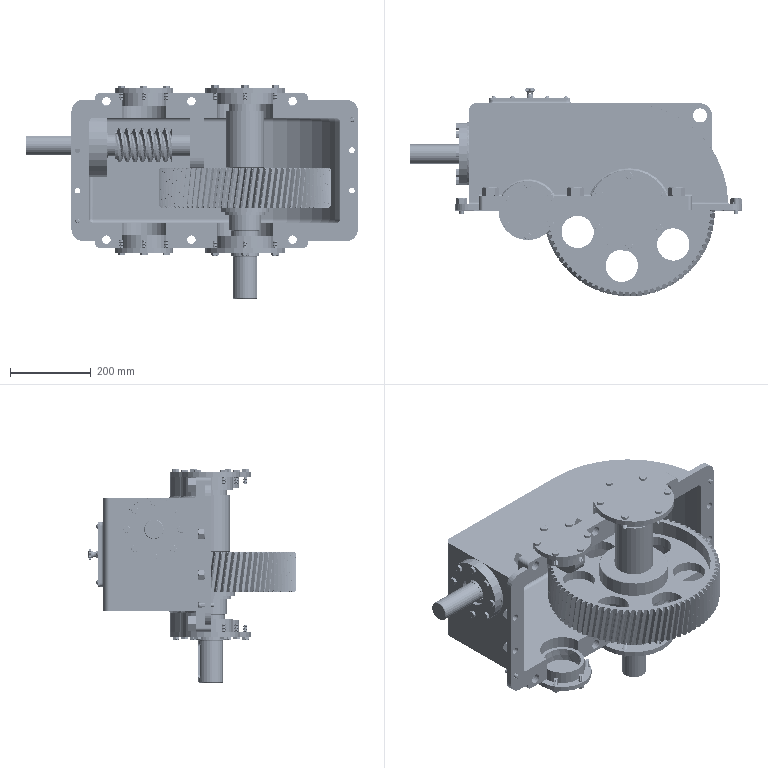Assembly | SolidWorks | mm | 84 component files | 84 solids | 4890 faces | box 820.25 x 516.08 x 527.4 mm | volume 19904523 mm3 | cylinder 2303 | plane 1060 | cone 558 | spline 498 | torus 360 | sphere 111 | commonest cylinder face diameters 10 x1442 0.5 x153 25 x112 20.75 x96 424.15 x83 6.708 x48 13 x27 11 x24
Bill of materials:
M10-30Bolt1 | 24 |  | Hex-head bolt-like part: hexagonal head with a short plain neck/undercut, then a long cylindrical shank with helical thread form to a flat end.
m16 | 4 |  | Tall hexagonal nut-like body with a central round through-bore and chamfered (arc-edged) hex corners at both ends.
M24 | 6 |  | Tall hexagonal nut-like body with a central threaded through-bore and chamfered hex corners at both ends.
FlangeOnLowSpeedAxis1 | 1 |  | Solid circular plate/blind flange with six through-holes on a bolt circle and a smaller-diameter raised cylindrical spigot on one face; no center bore.
FlangeOnLowSpeedAxis2 | 1 |  | Annular flange with six bolt holes and a raised cylindrical collar; the collar has a counterbore and a smaller central through-bore, forming an internal step.
FlangeOnWormWheelAxis | 2 |  | Cup-shaped flanged part: circular flange with six bolt holes supporting a tall cylindrical wall that encloses a recess with a closed bottom.
InvoluteLargeGear | 1 | Brass | Helical spur-type gear with many fine teeth, a recessed web containing six round lightening holes, a raised central hub, and a keyed central bore.
KeyOnLargeGear | 1 | Plain Carbon Steel | Small rectangular bar with fully rounded ends (obround/stadium plan shape) and small edge chamfers, resembling a round-ended parallel key.
LowSpeedAxis | 1 |  | Stepped cylindrical shaft with several coaxial diameter steps, largest step near one end with a short smaller pilot at that end, decreasing in diameter toward the other end.
SleeveOnLowSpeedAxis | 1 |  | Flat ring/washer with a stepped outer profile: a wider thin ring plus a slightly smaller-diameter thin step on one face, with a large central bore and small edge chamfers.
tapered roller bearings gb | 4 |  | Rolling-element bearing-like assembly: outer ring, inner ring and a single row of cylindrical rollers between them; inner ring protrudes axially on one side.
TaperPin | 2 |  | Solid tapered cylindrical pin, slightly larger diameter at one end, with chamfered edges at both ends.
circlips for holes--type a gb | 1 |  | Flat, thin open ring (C-shape) with uniform thickness. The two free ends widen into lugs, and each lug has a small round through-hole. Its form matches an internal-style retaining ring with lug holes.
FlangeOnWormAxis | 1 |  | Circular flat flange disc with a large central bore. It has eight equally spaced through-holes on a bolt circle and a short raised annular boss or face around the bore on one side.
hexagon socket button head screws gb | 6 |  | Solid pin with a domed (round) head and a plain cylindrical shank with a flat end. It has the shape of a solid round-head rivet blank.
M10-45 | 8 |  | Hex-head bolt. The shank is partly threaded, with a plain unthreaded section near the head and a short reduced-diameter neck directly under the head.
PeepHoleCover | 1 |  | Thin flat rectangular plate with rounded corners and nine through-holes: three across the top, three across the bottom, two at the mid-height side edges and one at the centre.
UpperHousing | 1 |  | Hollow, open-topped box-like housing with a perimeter mounting flange. Two side walls each have two semicircular bore cutouts with small holes around them, one end wall is curved, there is a rectangular opening with four holes in the floor, and an external lug has a single hole.
VentCap | 1 |  | Turned knob. It has a knurled, domed-top head, a concave waisted neck with a transverse cross-hole, a short collar and a smaller cylindrical spigot with a small axial bore at the end.
BearingSleeveOnWormAxis | 1 |  | Flanged tubular sleeve: a thin flat circular flange with eight equally spaced holes, joined to a short thin-walled cylindrical tube with a slight chamfer at its free end.
BearingInnerRing | 1 |  | Thick cylindrical ring or bush with a single external circumferential groove of rounded (concave) profile at about mid-width, and a plain cylindrical bore.
BearingOuterRing | 1 |  | Plain thin-walled cylindrical ring or band with slightly rounded or chamfered edges and a large bore.
Cage | 1 |  | Circular array of about 14 short ring-shaped loops, each joined to the next by small straight bar segments, forming a closed band.
RollingElement | 12 |  | Plain solid sphere.
WormAxis | 1 |  | Stepped cylindrical shaft with a short section of coarse helical thread (worm-like) between a long plain shank on one end and a short stepped journal on the other end.
Mates:
1. coincident | assembly face at (745.83, 1268.591, 1772.217) dir (0, 1, 0) | UpperHousingAssembly-1/UpperHousing-1 face at (890.83, 1268.591, 1632.217) dir (0, -1, 0)
2. concentric | assembly face at (798.33, 1008.59, 1803.217) dir (0, 1, 0) r 12.5 | UpperHousingAssembly-1/UpperHousing-1 face at (798.33, 1268.591, 1803.217) dir (0, 1, 0) r 12.5
3. concentric | UpperHousingAssembly-1/UpperHousing-1 face at (726.83, 1533.591, 1507.217) dir (0, -1, 0) r 6 | TaperPin-1 face at (726.83, 1299.341, 1507.217) dir (0, -1, 0) r 34.907
4. distance | TaperPin-1 face at (726.83, 1299.341, 1507.217) dir (0, 1, 0) | UpperHousingAssembly-1/UpperHousing-1 face at (890.83, 1283.591, 1632.217) dir (0, 1, 0)
5. concentric | UpperHousingAssembly-1/UpperHousing-1 face at (1404.83, 1533.591, 1757.217) dir (0, -1, 0) r 6 | TaperPin-2 face at (1404.83, 1299.341, 1757.217) dir (0, -1, 0) r 34.907
6. distance | TaperPin-2 face at (1404.83, 1299.341, 1757.217) dir (0, 1, 0) | UpperHousingAssembly-1/UpperHousing-1 face at (890.83, 1283.591, 1632.217) dir (0, 1, 0)
7. coincident | UpperHousingAssembly-1/UpperHousing-1 face at (890.83, 1303.591, 1632.217) dir (0, 1, 0) | M24-2 face at (1008.33, 1303.591, 1803.217) dir (0, -1, 0)
8. concentric | assembly face at (1258.33, 1008.59, 1461.217) dir (0, 1, 0) r 12.5 | assembly face at (798.33, 1453.938, 1461.217) dir (0, -1, 0) r 12
9. parallel | assembly face at (798.33, 1008.59, 1461.217) dir (0, 1, 0) r 12.5 | assembly face at (798.33, 1453.938, 1461.217) dir (0, -1, 0) r 12
10. concentric | assembly face at (798.33, 1008.59, 1461.217) dir (0, 1, 0) r 12.5 | assembly face at (798.33, 1453.938, 1461.217) dir (0, -1, 0) r 12
11. coincident | UpperHousingAssembly-1/UpperHousing-1 face at (890.83, 1303.591, 1632.217) dir (0, 1, 0) | M24-4 face at (1258.33, 1303.591, 1803.217) dir (0, -1, 0)
12. coincident | UpperHousingAssembly-1/UpperHousing-1 face at (890.83, 1303.591, 1632.217) dir (0, 1, 0) | M24-5 face at (798.33, 1303.591, 1461.217) dir (0, -1, 0)
13. coincident | UpperHousingAssembly-1/UpperHousing-1 face at (890.83, 1303.591, 1632.217) dir (0, 1, 0) | M24-7 face at (1258.33, 1303.591, 1461.217) dir (0, -1, 0)
14. coincident | UpperHousingAssembly-1/UpperHousing-1 face at (890.83, 1303.591, 1632.217) dir (0, 1, 0) | M24-6 face at (1008.33, 1303.591, 1461.217) dir (0, -1, 0)
15. concentric | PartAssemblyInLowerHousing-1/FlangeOnLowSpeedAxis2-1 face at (1140.83, 1354.591, 1428.217) dir (0, 0, 1) r 6.5 | M10-30Bolt1-1 face at (1140.83, 1354.591, 1458.217) dir (0, 0, 1) r 3.354
16. coincident | PartAssemblyInLowerHousing-1/FlangeOnLowSpeedAxis2-1 face at (1140.83, 1268.591, 1428.217) dir (0, 0, -1) | M10-30Bolt1-1 face at (1140.83, 1354.591, 1428.217) dir (0, 0, 1)
17. concentric | PartAssemblyInLowerHousing-1/FlangeOnWormWheelAxis-1 face at (890.83, 1332.591, 1429.217) dir (0, 0, 1) r 5.5 | M10-30Bolt1-7 face at (890.83, 1332.591, 1459.217) dir (0, 0, 1) r 3.354
18. coincident | PartAssemblyInLowerHousing-1/FlangeOnWormWheelAxis-1 face at (890.83, 1268.591, 1429.217) dir (0, 0, -1) | M10-30Bolt1-7 face at (890.83, 1332.591, 1429.217) dir (0, 0, 1)
19. concentric | PartAssemblyInLowerHousing-1/FlangeOnLowSpeedAxis1-1 face at (1140.83, 1354.591, 1797.467) dir (0, 0, 1) r 6.5 | M10-30Bolt1-13 face at (1140.83, 1354.591, 1806.217) dir (0, 0, -1) r 3.354
20. coincident | PartAssemblyInLowerHousing-1/FlangeOnLowSpeedAxis1-1 face at (1054.227, 1318.591, 1836.217) dir (0, 0, 1) | M10-30Bolt1-13 face at (1140.83, 1354.591, 1836.217) dir (0, 0, -1)
21. concentric | PartAssemblyInLowerHousing-1/FlangeOnWormWheelAxis-2 face at (890.83, 1332.591, 1835.217) dir (0, 0, -1) r 5.5 | M10-30Bolt1-25 face at (890.83, 1332.591, 1805.217) dir (0, 0, -1) r 3.354
22. coincident | PartAssemblyInLowerHousing-1/FlangeOnWormWheelAxis-2 face at (890.83, 1268.591, 1835.217) dir (0, 0, 1) | M10-30Bolt1-25 face at (890.83, 1332.591, 1835.217) dir (0, 0, -1)
23. coincident | UpperHousingAssembly-1/UpperHousing-1 face at (890.83, 1283.591, 1632.217) dir (0, 1, 0) | m16-2 face at (726.83, 1283.591, 1582.217) dir (0, -1, 0)
24. coincident | UpperHousingAssembly-1/UpperHousing-1 face at (890.83, 1283.591, 1632.217) dir (0, 1, 0) | m16-3 face at (726.83, 1283.591, 1682.217) dir (0, -1, 0)
25. coincident | UpperHousingAssembly-1/UpperHousing-1 face at (890.83, 1283.591, 1632.217) dir (0, 1, 0) | m16-4 face at (1404.83, 1283.591, 1682.217) dir (0, -1, 0)
26. coincident | UpperHousingAssembly-1/UpperHousing-1 face at (890.83, 1283.591, 1632.217) dir (0, 1, 0) | m16-5 face at (1404.83, 1283.591, 1582.217) dir (0, -1, 0)
27. concentric | LowSpeedAxisAssembly-1/tapered roller bearings gb-4 face at (1221.289, 1355.939, 1464.523) dir (0, 0, -1) r 32.5 | FlangeOnLowSpeedAxis1-1 face at (1221.289, 1355.939, 1508.526) dir (0, 0, 1) r 34.907
28. coincident | LowSpeedAxisAssembly-1/tapered roller bearings gb-4 face at (1192.973, 1369.74, 1482.776) dir (0, 0, 1) | FlangeOnLowSpeedAxis1-1 face at (1167.596, 1386.939, 1482.776) dir (0, 0, -1)
29. coincident | LowSpeedAxis-1 face at (1124.62, 1130.298, 1182.59) dir (0, 1, 0) | KeyOnLargeGear-1 face at (1059.62, 1130.298, 1182.59) dir (0, -1, 0)
30. concentric | LowSpeedAxis-1 face at (1124.62, 1130.298, 1182.59) dir (0, 1, 0) r 11 | KeyOnLargeGear-1 face at (1124.62, 1130.298, 1182.59) dir (0, 1, 0) r 11
31. coincident | KeyOnLargeGear-1 face at (1059.62, 1130.298, 1193.59) dir (0, 0, 1) | InvoluteLargeGear-1 face at (1139.626, 1137.849, 1193.59) dir (0, 0, -1)
32. coincident | LowSpeedAxis-1 face at (1139.62, 1139.298, 1182.59) dir (-1, 0, 0) | InvoluteLargeGear-1 face at (1139.62, 1096.798, 1182.59) dir (1, 0, 0)
33. concentric | LowSpeedAxis-1 face at (805.297, 1096.798, 1182.59) dir (-1, 0, 0) r 40 | SleeveOnLowSpeedAxis-1 face at (1039.62, 1096.798, 1182.59) dir (1, 0, 0) r 40
34. coincident | InvoluteLargeGear-1 face at (1039.62, 1096.798, 1182.59) dir (-1, 0, 0) | SleeveOnLowSpeedAxis-1 face at (1039.62, 1087.814, 1241.914) dir (1, 0, 0)
35. concentric | LowSpeedAxis-1 face at (805.297, 1096.798, 1182.59) dir (-1, 0, 0) r 40 | tapered roller bearings gb-3 face at (1021.87, 1096.798, 1182.59) dir (1, 0, 0) r 16
36. coincident | SleeveOnLowSpeedAxis-1 face at (1021.87, 1090.809, 1222.139) dir (-1, 0, 0) | tapered roller bearings gb-3 face at (1021.87, 1096.798, 1182.59) dir (1, 0, 0)
37. concentric | LowSpeedAxis-1 face at (805.297, 1096.798, 1182.59) dir (-1, 0, 0) r 40 | tapered roller bearings gb-4 face at (1279.62, 1096.798, 1182.59) dir (-1, 0, 0) r 16
38. coincident | LowSpeedAxis-1 face at (1279.62, 1144.298, 1182.59) dir (1, 0, 0) | tapered roller bearings gb-4 face at (1279.62, 1096.798, 1182.59) dir (-1, 0, 0)
39. concentric | LowSpeedAxis-1 face at (805.297, 1096.798, 1182.59) dir (-1, 0, 0) r 42.5 | InvoluteLargeGear-1 face at (1139.626, 1096.798, 1182.59) dir (-1, 0, 0) r 42.5
40. concentric | UpperHousing-1 face at (835.485, 1282.284, 1275.253) dir (1, 0, 0) r 50 | circlips for holes--type a gb-1 face at (1154.736, 1282.284, 1275.253) dir (1, 0, 0) r 6.5
41. coincident | UpperHousing-1 face at (1154.736, 1282.284, 1328.003) dir (1, 0, 0) | circlips for holes--type a gb-1 face at (1154.736, 1282.284, 1275.253) dir (-1, 0, 0)
42. concentric | UpperHousing-1 face at (864.486, 1282.284, 1275.253) dir (-1, 0, 0) r 55 | WormAxisAssembly-1/BearingSleeveOnWormAxis-1 face at (920.486, 1282.284, 1275.253) dir (-1, 0, 0) r 55
43. concentric | UpperHousing-1 face at (864.486, 1349.284, 1275.253) dir (-1, 0, 0) r 5 | WormAxisAssembly-1/BearingSleeveOnWormAxis-1 edge at (855.486, 1349.284, 1275.253) dir (-1, 0, 0) r 5.275
44. coincident | UpperHousing-1 face at (864.486, 1282.284, 1275.253) dir (-1, 0, 0) | WormAxisAssembly-1/BearingSleeveOnWormAxis-1 face at (864.486, 1282.284, 1275.253) dir (1, 0, 0)
45. coincident | WormAxisAssembly-1/BearingSleeveOnWormAxis-1 face at (855.486, 1282.284, 1275.253) dir (-1, 0, 0) | FlangeOnWormAxis-1 face at (855.486, 1360.284, 1275.253) dir (1, 0, 0)
46. concentric | WormAxisAssembly-1/WormAxis-1 face at (723.233, 1282.284, 1275.253) dir (-1, 0, 0) r 24 | FlangeOnWormAxis-1 face at (843.486, 1282.284, 1275.253) dir (-1, 0, 0) r 78
47. concentric | UpperHousing-1 face at (864.486, 1329.66, 1322.629) dir (-1, 0, 0) r 5 | FlangeOnWormAxis-1 face at (861.986, 1329.66, 1322.629) dir (-1, 0, 0) r 5.25
48. coincident | UpperHousing-1 face at (1014.486, 1415.284, 1213.253) dir (0, 1, 0) | PeepHoleCover-1 face at (1019.486, 1415.284, 1213.253) dir (0, -1, 0)
49. concentric | UpperHousing-1 edge at (1061.986, 1415.284, 1282.253) dir (0, 1, 0) r 5 | PeepHoleCover-1 edge at (1061.986, 1421.284, 1282.253) dir (0, 1, 0) r 5
50. concentric | UpperHousing-1 edge at (930.486, 1415.284, 1213.253) dir (0, 1, 0) r 5 | PeepHoleCover-1 edge at (930.486, 1421.284, 1213.253) dir (0, 1, 0) r 5
51. concentric | PeepHoleCover-1 face at (1019.486, 1421.284, 1213.253) dir (0, 1, 0) r 5 | VentCap-1 face at (1019.486, 1411.284, 1213.253) dir (0, -1, 0) r 5
52. coincident | PeepHoleCover-1 face at (1019.486, 1421.284, 1213.253) dir (0, 1, 0) | VentCap-1 edge at (1019.486, 1421.284, 1213.253) dir (0, -1, 0) r 8
53. concentric | FlangeOnWormAxis-1 face at (861.986, 1349.284, 1275.253) dir (-1, 0, 0) r 5.25 | M10-45-1 face at (888.486, 1349.284, 1275.253) dir (1, 0, 0) r 3.092
54. coincident | FlangeOnWormAxis-1 face at (843.486, 1318.284, 1275.253) dir (-1, 0, 0) | M10-45-1 face at (843.486, 1349.284, 1275.253) dir (1, 0, 0)
55. concentric | FlangeOnWormAxis-1 face at (861.986, 1329.66, 1227.877) dir (-1, 0, 0) r 5.25 | M10-45-3 face at (888.486, 1329.66, 1227.877) dir (1, 0, 0) r 3.092
56. concentric | FlangeOnWormAxis-1 face at (861.986, 1282.284, 1208.253) dir (-1, 0, 0) r 5.25 | M10-45-6 face at (888.486, 1282.284, 1208.253) dir (1, 0, 0) r 3.092
57. concentric | FlangeOnWormAxis-1 edge at (843.486, 1329.66, 1322.629) dir (-1, 0, 0) r 5.25 | M10-45-7 face at (888.486, 1329.66, 1322.629) dir (1, 0, 0) r 3.092
58. concentric | FlangeOnWormAxis-1 face at (861.986, 1282.284, 1342.253) dir (-1, 0, 0) r 5.25 | M10-45-2 face at (888.486, 1282.284, 1342.253) dir (1, 0, 0) r 3.092
59. concentric | FlangeOnWormAxis-1 face at (861.986, 1234.908, 1227.877) dir (-1, 0, 0) r 5.25 | M10-45-4 face at (888.486, 1234.908, 1227.877) dir (1, 0, 0) r 3.092
60. concentric | FlangeOnWormAxis-1 face at (861.986, 1215.284, 1275.253) dir (-1, 0, 0) r 5.25 | M10-45-5 face at (888.486, 1215.284, 1275.253) dir (1, 0, 0) r 3.092
61. concentric | FlangeOnWormAxis-1 face at (861.986, 1234.908, 1322.629) dir (-1, 0, 0) r 5.25 | M10-45-8 face at (888.486, 1234.908, 1322.629) dir (1, 0, 0) r 3.092
62. coincident | FlangeOnWormAxis-1 face at (843.486, 1318.284, 1275.253) dir (-1, 0, 0) | M10-45-8 face at (843.486, 1234.908, 1322.629) dir (1, 0, 0)
63. coincident | FlangeOnWormAxis-1 face at (843.486, 1318.284, 1275.253) dir (-1, 0, 0) | M10-45-4 face at (843.486, 1234.908, 1227.877) dir (1, 0, 0)
64. coincident | FlangeOnWormAxis-1 face at (843.486, 1318.284, 1275.253) dir (-1, 0, 0) | M10-45-5 face at (843.486, 1215.284, 1275.253) dir (1, 0, 0)
65. coincident | FlangeOnWormAxis-1 face at (843.486, 1318.284, 1275.253) dir (-1, 0, 0) | M10-45-3 face at (843.486, 1329.66, 1227.877) dir (1, 0, 0)
66. coincident | FlangeOnWormAxis-1 face at (843.486, 1318.284, 1275.253) dir (-1, 0, 0) | M10-45-6 face at (843.486, 1282.284, 1208.253) dir (1, 0, 0)
67. coincident | FlangeOnWormAxis-1 face at (843.486, 1318.284, 1275.253) dir (-1, 0, 0) | M10-45-7 face at (843.486, 1329.66, 1322.629) dir (1, 0, 0)
68. coincident | FlangeOnWormAxis-1 face at (843.486, 1318.284, 1275.253) dir (-1, 0, 0) | M10-45-2 face at (843.486, 1282.284, 1342.253) dir (1, 0, 0)
69. concentric | PeepHoleCover-1 face at (1061.986, 1421.284, 1282.253) dir (0, 1, 0) r 5 | hexagon socket button head screws gb-8 face at (1061.986, 1401.284, 1282.253) dir (0, 1, 0) r 3
70. coincident | PeepHoleCover-1 face at (1019.486, 1421.284, 1213.253) dir (0, 1, 0) | hexagon socket button head screws gb-8 face at (1061.986, 1421.284, 1282.253) dir (0, -1, 0)
71. concentric | PeepHoleCover-1 face at (976.986, 1421.284, 1282.253) dir (0, 1, 0) r 5 | hexagon socket button head screws gb-9 face at (976.986, 1401.284, 1282.253) dir (0, 1, 0) r 3
72. coincident | PeepHoleCover-1 face at (1019.486, 1421.284, 1213.253) dir (0, 1, 0) | hexagon socket button head screws gb-9 face at (976.986, 1421.284, 1282.253) dir (0, -1, 0)
73. concentric | PeepHoleCover-1 face at (930.486, 1421.284, 1213.253) dir (0, 1, 0) r 5 | hexagon socket button head screws gb-10 face at (930.486, 1401.284, 1213.253) dir (0, 1, 0) r 3
74. coincident | PeepHoleCover-1 face at (1019.486, 1421.284, 1213.253) dir (0, 1, 0) | hexagon socket button head screws gb-10 face at (930.486, 1421.284, 1213.253) dir (0, -1, 0)
75. concentric | PeepHoleCover-1 face at (976.986, 1421.284, 1144.253) dir (0, 1, 0) r 5 | hexagon socket button head screws gb-11 face at (976.986, 1401.284, 1144.253) dir (0, 1, 0) r 3
76. coincident | PeepHoleCover-1 face at (1019.486, 1421.284, 1213.253) dir (0, 1, 0) | hexagon socket button head screws gb-11 face at (976.986, 1421.284, 1144.253) dir (0, -1, 0)
77. concentric | PeepHoleCover-1 face at (1061.986, 1421.284, 1144.253) dir (0, 1, 0) r 5 | hexagon socket button head screws gb-12 face at (1061.986, 1401.284, 1144.253) dir (0, 1, 0) r 3
78. coincident | PeepHoleCover-1 face at (1019.486, 1421.284, 1213.253) dir (0, 1, 0) | hexagon socket button head screws gb-12 face at (1061.986, 1421.284, 1144.253) dir (0, -1, 0)
79. concentric | PeepHoleCover-1 face at (1108.486, 1421.284, 1213.253) dir (0, 1, 0) r 5 | hexagon socket button head screws gb-13 face at (1108.486, 1401.284, 1213.253) dir (0, 1, 0) r 3
80. coincident | PeepHoleCover-1 face at (1019.486, 1421.284, 1213.253) dir (0, 1, 0) | hexagon socket button head screws gb-13 face at (1108.486, 1421.284, 1213.253) dir (0, -1, 0)
81. concentric | WormAxis-1 face at (855.062, 1105.253, 1134.051) dir (-1, 0, 0) r 22.5 | DeepGrooveBallBearing6309-1/BearingInnerRing-1 face at (1255.642, 1105.253, 1134.051) dir (-1, 0, 0) r 22.5
82. coincident | WormAxis-1 face at (1262.062, 1132.753, 1134.051) dir (1, 0, 0) | DeepGrooveBallBearing6309-1/BearingInnerRing-1 face at (1262.062, 1127.753, 1134.051) dir (-1, 0, 0)
83. concentric | tapered roller bearings gb-3 face at (1029.062, 1105.253, 1134.051) dir (-1, 0, 0) r 32.5 | tapered roller bearings gb-4 face at (1029.062, 1105.253, 1134.051) dir (1, 0, 0) r 32.5
84. coincident | tapered roller bearings gb-3 face at (1029.062, 1105.253, 1134.051) dir (-1, 0, 0) | tapered roller bearings gb-4 face at (1029.062, 1105.253, 1134.051) dir (1, 0, 0)
85. concentric | BearingSleeveOnWormAxis-1 face at (1047.315, 1105.253, 1134.051) dir (-1, 0, 0) r 50 | tapered roller bearings gb-4 face at (1029.062, 1105.253, 1134.051) dir (1, 0, 0) r 32.5
86. coincident | BearingSleeveOnWormAxis-1 face at (1047.315, 1105.253, 1134.051) dir (-1, 0, 0) | tapered roller bearings gb-3 face at (1047.315, 1135.278, 1143.576) dir (1, 0, 0)
87. concentric | WormAxis-1 face at (855.062, 1105.253, 1134.051) dir (-1, 0, 0) r 27.5 | BearingSleeveOnWormAxis-1 face at (1052.315, 1105.253, 1134.051) dir (-1, 0, 0) r 55
88. coincident | WormAxis-1 face at (1046.062, 1132.753, 1134.051) dir (-1, 0, 0) | tapered roller bearings gb-3 face at (1046.062, 1105.253, 1134.051) dir (1, 0, 0)
89. concentric | BearingInnerRing-1 face at (1013.335, 1022.594, 1021.051) dir (-1, 0, 0) r 22.5 | BearingOuterRing-1 face at (1026.403, 1022.594, 1021.051) dir (-1, 0, 0) r 50
90. coincident | BearingInnerRing-1 face at (1044.754, 1045.094, 1021.051) dir (1, 0, 0) | BearingOuterRing-1 face at (1044.754, 1072.594, 1021.051) dir (1, 0, 0)
91. coincident | BearingOuterRing-1 plane at (1032.254, 1022.594, 1021.051) dir (1, 0, 0) | Cage-1 plane at (1032.254, 1022.594, 1021.051) dir (1, 0, 0)
92. coincident | BearingInnerRing-1 axis at (1044.754, 1022.594, 1021.051) dir (-1, 0, 0) | Cage-1 axis at (1031.254, 1022.594, 1021.051) dir (1, 0, 0)
93. concentric | RollingElement-1 face at (1032.254, 1055.661, 1006.197) dir (1, 0, 0) r 6.85 | Cage-1 face at (1032.254, 1055.661, 1006.197) dir (1, 0, 0) r 7.5